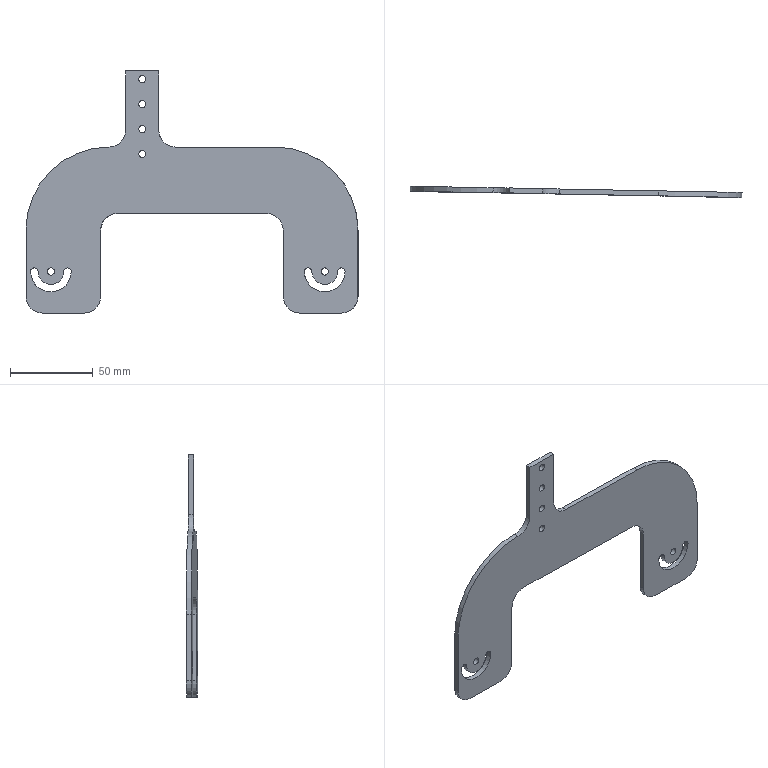Component | SolidWorks | DM17A08-02-002-1 | 1 solid | 43 faces | volume 38526 mm3 | cylinder 30 | plane 13 | commonest cylinder face diameters 4.3 x12 20 x8 4.5 x4 100 x2 15.5 x2 24.5 x2